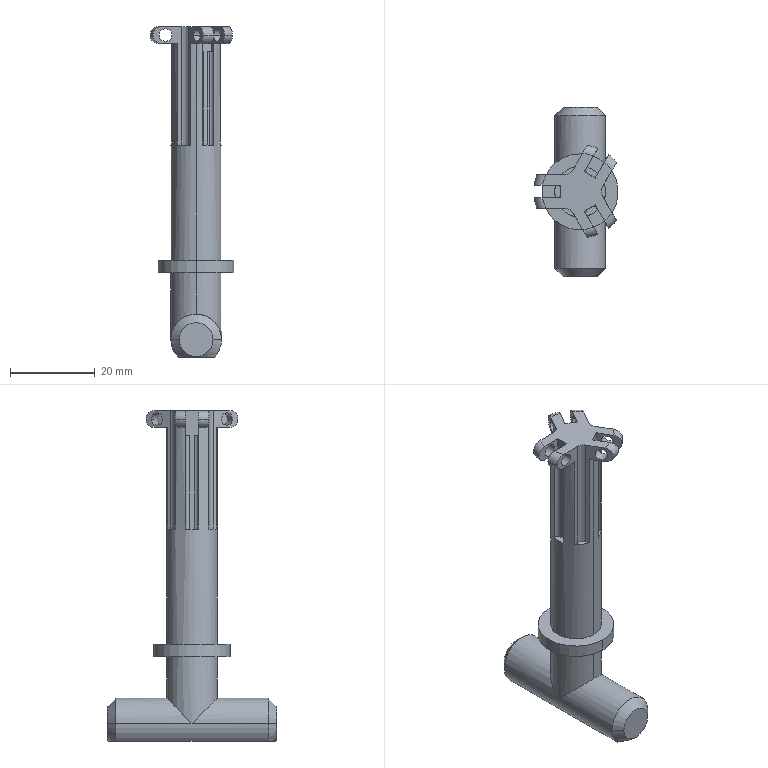Component | SolidWorks | g-1 | 1 solid | 87 faces | volume 11846 mm3 | plane 38 | cylinder 33 | torus 12 | cone 4 | commonest cylinder face diameters 3 x12 2 x8 12 x8 4 x3 18 x2